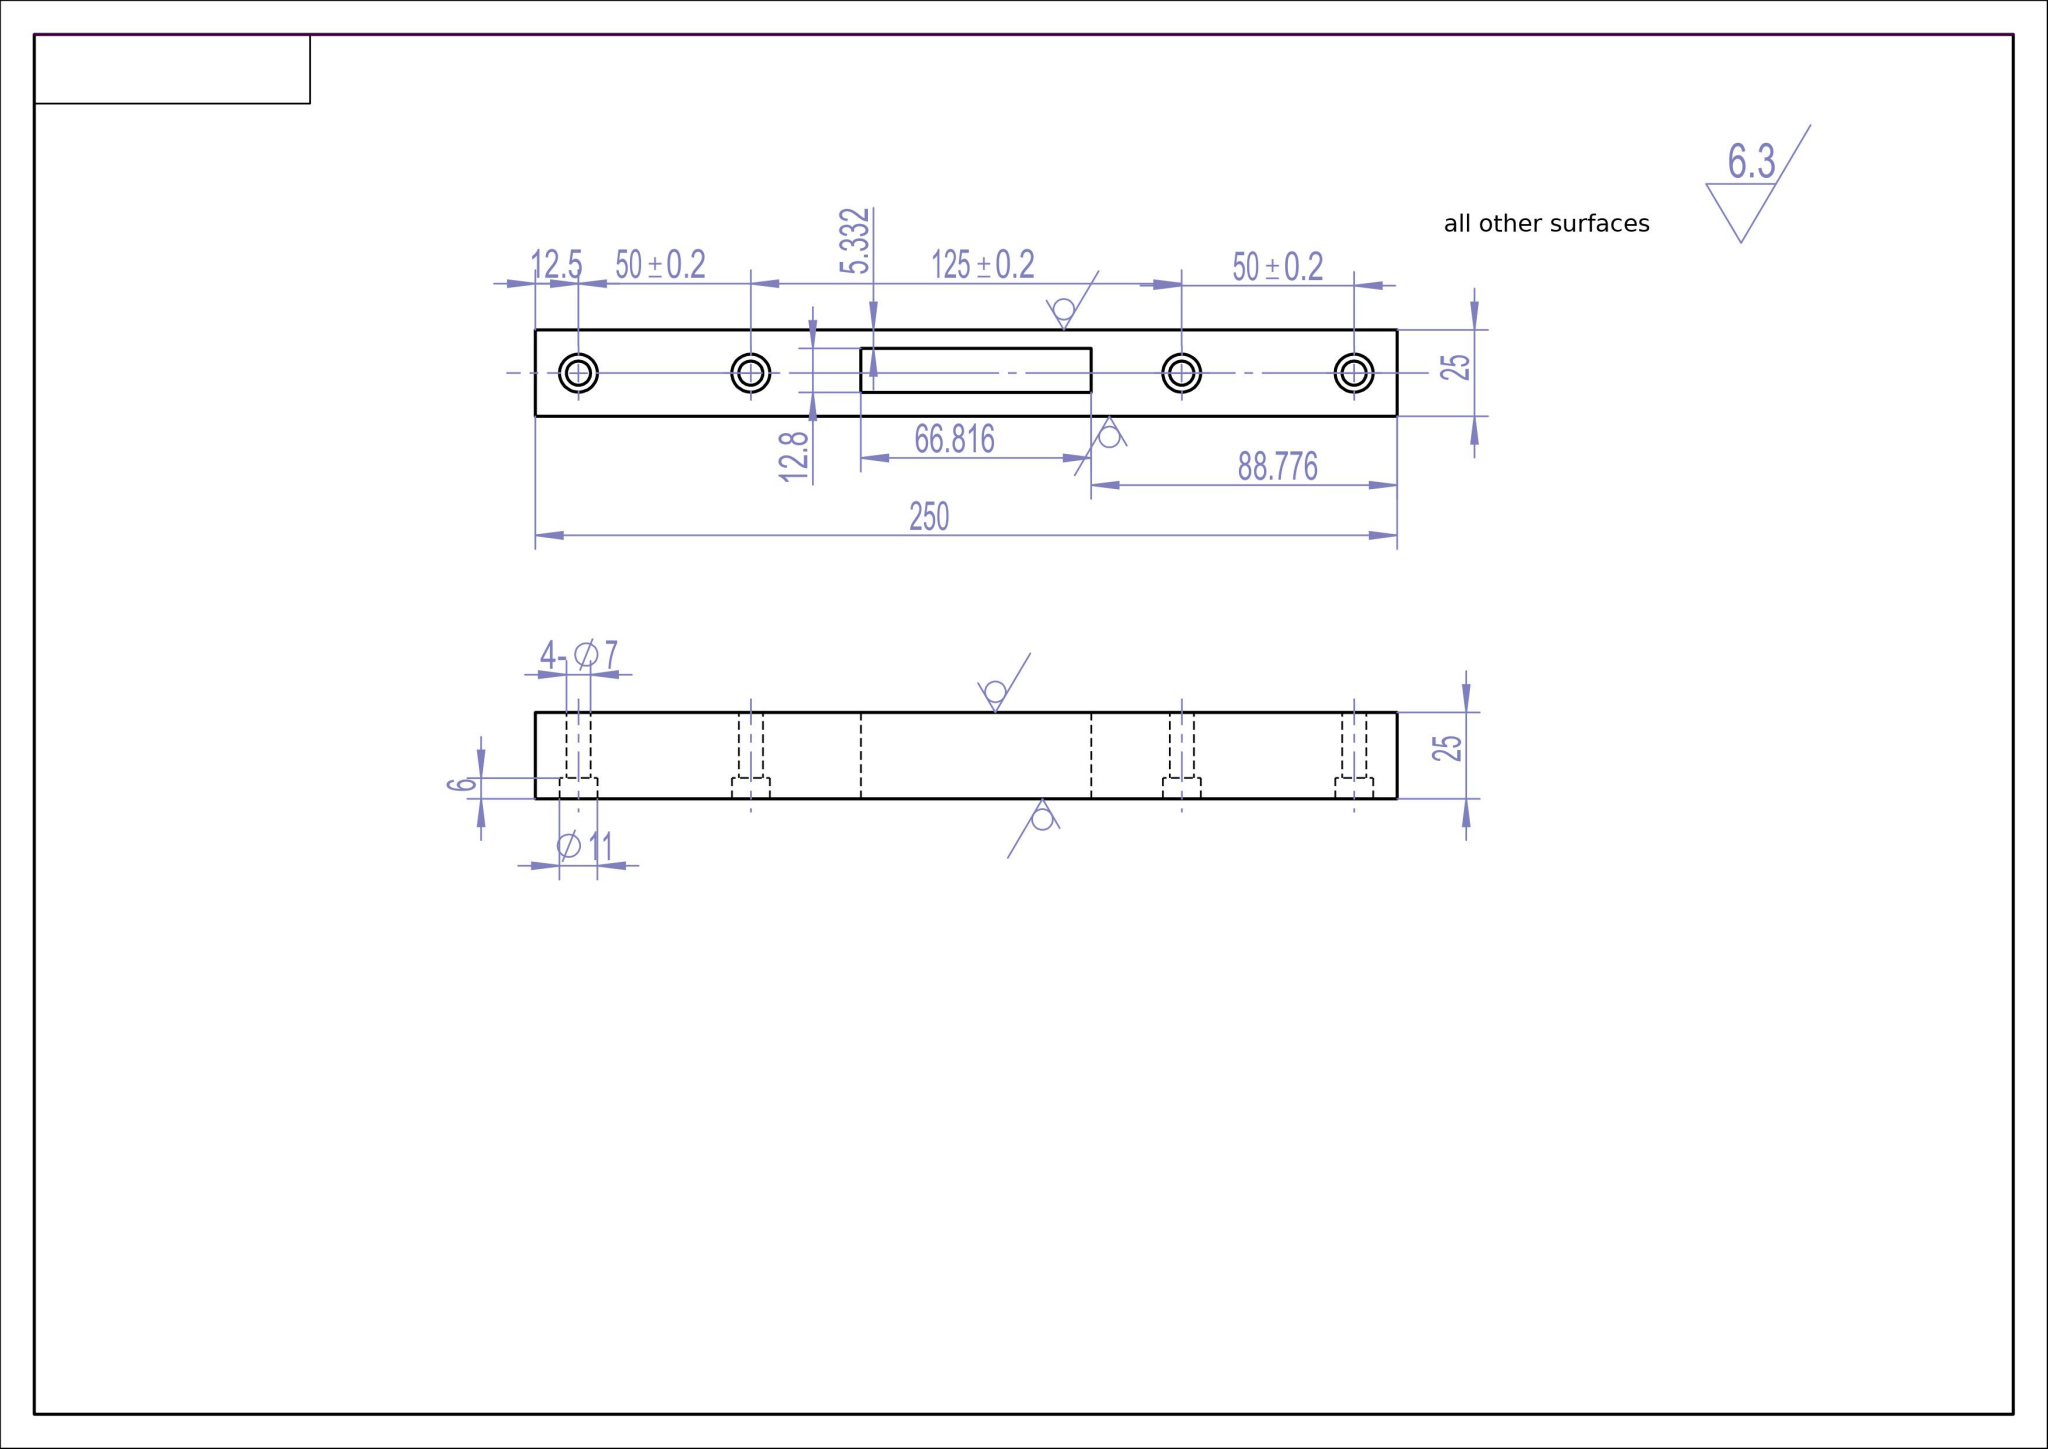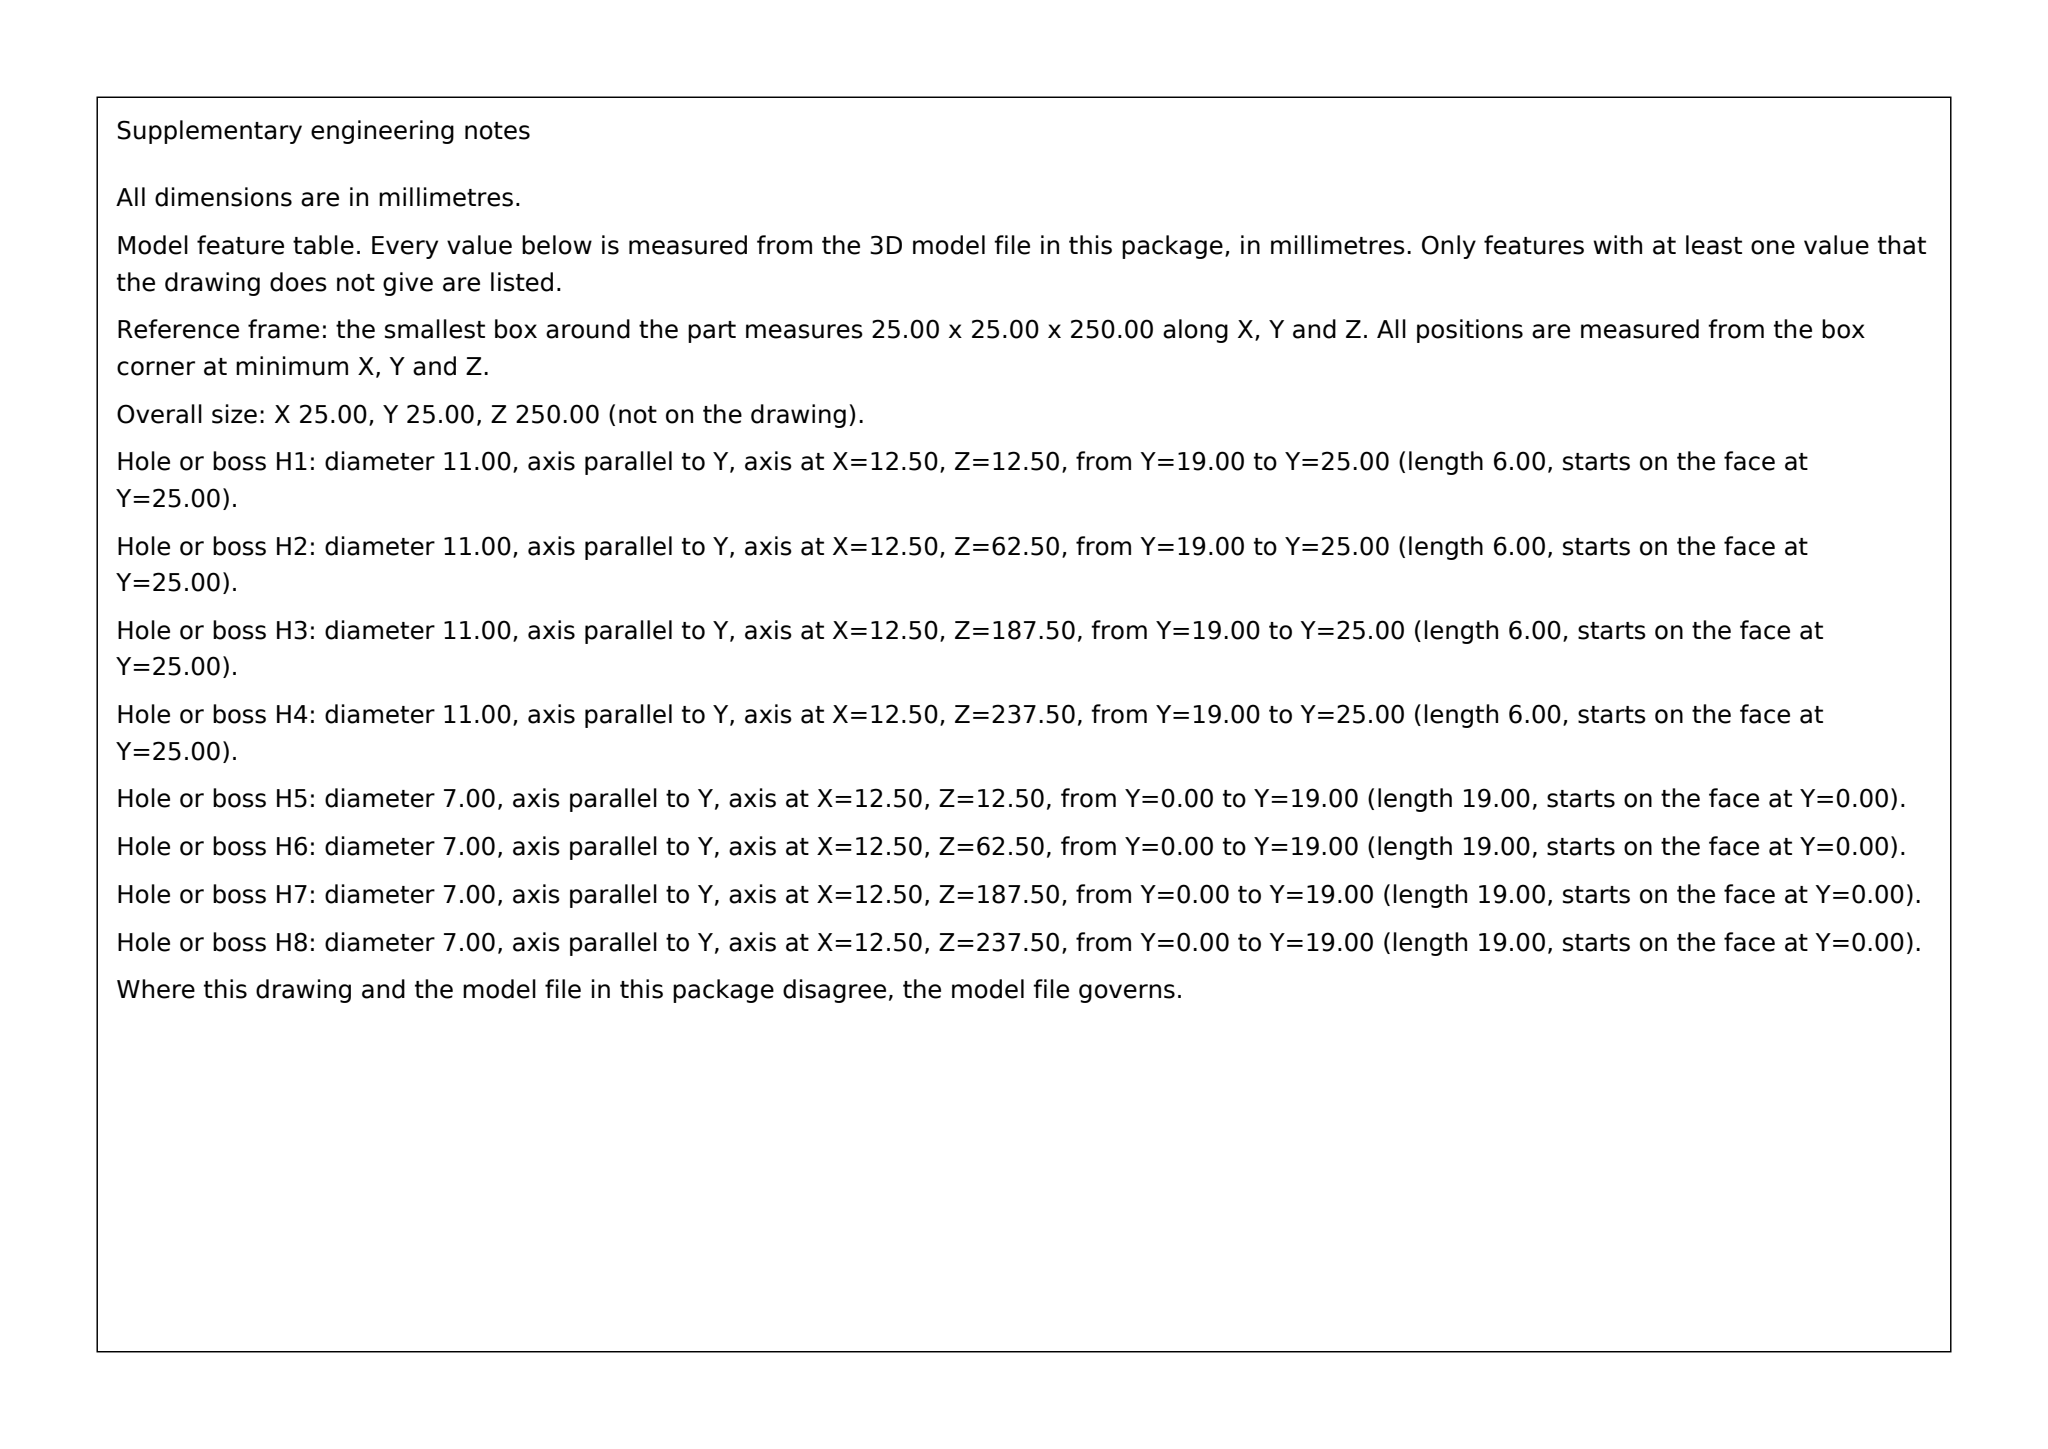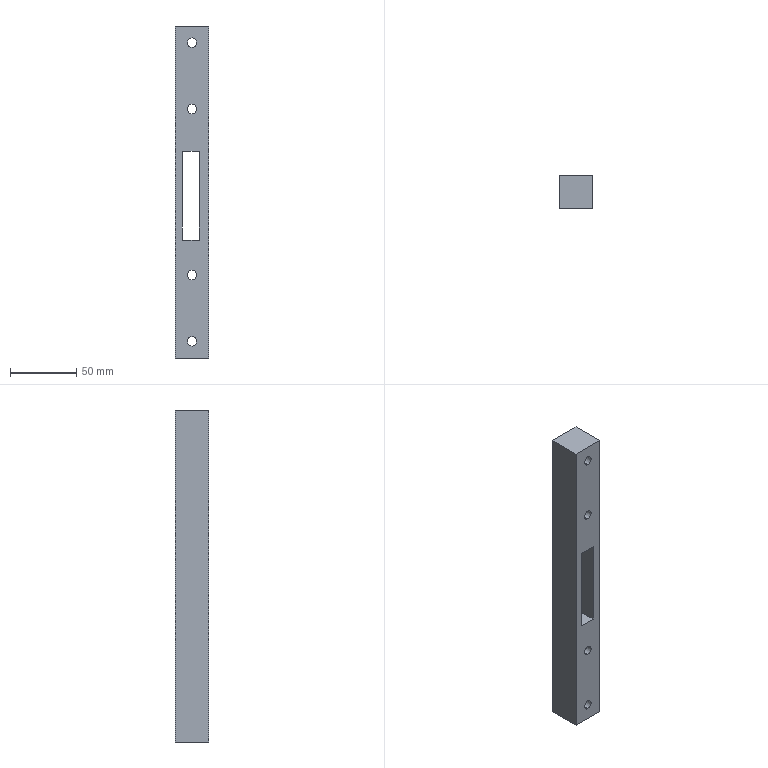Part | SolidWorks | mm | 1 solid | 30 faces | box 25 x 25 x 250 mm | volume 129663 mm3 | cylinder 16 | plane 14 | commonest cylinder face diameters 7 x8 11 x8
build123d program:
from build123d import *

# Parameters (mm, degrees)
SKETCH1_W                 = 25
SKETCH1_H                 = 25
BOSS_EXTRUDE1_DEPTH       = 250
SKETCH2_R                 = 5.5
CUT_EXTRUDE1_DEPTH        = 6
SKETCH3_R                 = 3.5
CUT_EXTRUDE2_DEPTH        = 26
LPATTERN1_COUNT           = 2
LPATTERN1_PITCH           = 50
LPATTERN2_COUNT           = 2
LPATTERN2_PITCH           = 175
LPATTERN2_COPY_1_SKETCH_R = 5.5
LPATTERN2_COPY_1_DEPTH    = 6
LPATTERN2_COPY_2_SKETCH_R = 3.5
LPATTERN2_COPY_2_DEPTH    = 26
SKETCH4_W                 = 12.8
SKETCH4_H                 = 66.816
CUT_EXTRUDE3_DEPTH        = 88


with BuildPart() as part:
    # Sketch1 → Boss-Extrude1 (new body)
    with BuildSketch(Plane.XY):
        with Locations((-44.867, 3.806)):
            Rectangle(SKETCH1_W, SKETCH1_H)
    extrude(amount=BOSS_EXTRUDE1_DEPTH)

    # Sketch2 → Cut-Extrude1 (cut)
    with BuildSketch(Plane(origin=(0, 16.306, 0), x_dir=(1, 0, 0), z_dir=(0, 1, 0))):
        with Locations(Location((-44.867, -12.5, 0), (0, 0, 270))):
            Circle(SKETCH2_R)
    cut_extrude1 = extrude(amount=-CUT_EXTRUDE1_DEPTH, mode=Mode.SUBTRACT)

    # Sketch3 → Cut-Extrude2 (cut)
    with BuildSketch(Plane(origin=(0, 10.306, 0), x_dir=(1, 0, 0), z_dir=(0, 1, 0))):
        with Locations(Location((-44.867, -12.5, 0), (0, 0, 270))):
            Circle(SKETCH3_R)
    cut_extrude2 = extrude(amount=-CUT_EXTRUDE2_DEPTH, mode=Mode.SUBTRACT)

    # LPattern1: Cut-Extrude1, Cut-Extrude2 ×2
    with Locations(*[(0, 0, i * LPATTERN1_PITCH) for i in range(1, LPATTERN1_COUNT)]):
        add(cut_extrude1, mode=Mode.SUBTRACT)
        add(cut_extrude2, mode=Mode.SUBTRACT)

    # LPattern2: Cut-Extrude1, Cut-Extrude2 ×2
    with Locations(*[(0, 0, i * LPATTERN2_PITCH) for i in range(1, LPATTERN2_COUNT)]):
        add(cut_extrude1, mode=Mode.SUBTRACT)
        add(cut_extrude2, mode=Mode.SUBTRACT)

    # LPattern2 copy 1 sketch → LPattern2 copy 1 (cut)
    with BuildSketch(Plane(origin=(0, 16.306, 225), x_dir=(1, 0, 0), z_dir=(0, 1, 0))):
        with Locations(Location((-44.867, -12.5, 0), (0, 0, 270))):
            Circle(LPATTERN2_COPY_1_SKETCH_R)
    extrude(amount=-LPATTERN2_COPY_1_DEPTH, mode=Mode.SUBTRACT)

    # LPattern2 copy 2 sketch → LPattern2 copy 2 (cut)
    with BuildSketch(Plane(origin=(0, 10.306, 225), x_dir=(1, 0, 0), z_dir=(0, 1, 0))):
        with Locations(Location((-44.867, -12.5, 0), (0, 0, 270))):
            Circle(LPATTERN2_COPY_2_SKETCH_R)
    extrude(amount=-LPATTERN2_COPY_2_DEPTH, mode=Mode.SUBTRACT)

    # Sketch4 → Cut-Extrude3 (cut)
    with BuildSketch(Plane(origin=(0, 16.306, 0), x_dir=(1, 0, 0), z_dir=(0, 1, 0))):
        with Locations((-45.635, -122.184)):
            Rectangle(SKETCH4_W, SKETCH4_H)
    extrude(amount=-CUT_EXTRUDE3_DEPTH, mode=Mode.SUBTRACT)


solid = part.part
STEP:
#1=CARTESIAN_POINT('',(-44.867,-8.694,234.));
#2=VERTEX_POINT('',#1);
#3=CARTESIAN_POINT('',(-44.867,-8.694,241.));
#4=VERTEX_POINT('',#3);
#5=CARTESIAN_POINT('',(-44.867,-8.694,237.5));
#6=DIRECTION('',(0.,1.,0.));
#7=DIRECTION('',(0.,0.,1.));
#8=AXIS2_PLACEMENT_3D('',#5,#6,#7);
#9=CIRCLE('',#8,3.5);
#10=EDGE_CURVE('',#2,#4,#9,.T.);
#11=ORIENTED_EDGE('',*,*,#10,.F.);
#12=CARTESIAN_POINT('',(-44.867,10.306,234.));
#13=VERTEX_POINT('',#12);
#14=CARTESIAN_POINT('',(-44.867,-15.694,234.));
#15=DIRECTION('',(0.,1.,0.));
#16=VECTOR('',#15,1000.);
#17=LINE('',#14,#16);
#18=EDGE_CURVE('',#2,#13,#17,.T.);
#19=ORIENTED_EDGE('',*,*,#18,.T.);
#20=CARTESIAN_POINT('',(-44.867,10.306,241.));
#21=VERTEX_POINT('',#20);
#22=CARTESIAN_POINT('',(-44.867,10.306,237.5));
#23=DIRECTION('',(0.,1.,0.));
#24=DIRECTION('',(0.,0.,1.));
#25=AXIS2_PLACEMENT_3D('',#22,#23,#24);
#26=CIRCLE('',#25,3.5);
#27=EDGE_CURVE('',#13,#21,#26,.T.);
#28=ORIENTED_EDGE('',*,*,#27,.T.);
#29=CARTESIAN_POINT('',(-44.867,-15.694,241.));
#30=DIRECTION('',(0.,1.,0.));
#31=VECTOR('',#30,1000.);
#32=LINE('',#29,#31);
#33=EDGE_CURVE('',#4,#21,#32,.T.);
#34=ORIENTED_EDGE('',*,*,#33,.F.);
#35=EDGE_LOOP('',(#11,#19,#28,#34));
#36=FACE_OUTER_BOUND('',#35,.T.);
#37=CARTESIAN_POINT('',(-44.867,-15.694,237.5));
#38=DIRECTION('',(0.,1.,0.));
#39=DIRECTION('',(0.,0.,1.));
#40=AXIS2_PLACEMENT_3D('',#37,#38,#39);
#41=CYLINDRICAL_SURFACE('',#40,3.5);
#42=ADVANCED_FACE('',(#36),#41,.F.);
#43=CARTESIAN_POINT('',(-44.867,-8.694,184.));
#44=VERTEX_POINT('',#43);
#45=CARTESIAN_POINT('',(-44.867,-8.694,191.));
#46=VERTEX_POINT('',#45);
#47=CARTESIAN_POINT('',(-44.867,-8.694,187.5));
#48=DIRECTION('',(0.,1.,0.));
#49=DIRECTION('',(0.,0.,1.));
#50=AXIS2_PLACEMENT_3D('',#47,#48,#49);
#51=CIRCLE('',#50,3.5);
#52=EDGE_CURVE('',#44,#46,#51,.T.);
#53=ORIENTED_EDGE('',*,*,#52,.F.);
#54=CARTESIAN_POINT('',(-44.867,10.306,184.));
#55=VERTEX_POINT('',#54);
#56=CARTESIAN_POINT('',(-44.867,-15.694,184.));
#57=DIRECTION('',(0.,1.,0.));
#58=VECTOR('',#57,1000.);
#59=LINE('',#56,#58);
#60=EDGE_CURVE('',#44,#55,#59,.T.);
#61=ORIENTED_EDGE('',*,*,#60,.T.);
#62=CARTESIAN_POINT('',(-44.867,10.306,191.));
#63=VERTEX_POINT('',#62);
#64=CARTESIAN_POINT('',(-44.867,10.306,187.5));
#65=DIRECTION('',(0.,1.,0.));
#66=DIRECTION('',(0.,0.,1.));
#67=AXIS2_PLACEMENT_3D('',#64,#65,#66);
#68=CIRCLE('',#67,3.5);
#69=EDGE_CURVE('',#55,#63,#68,.T.);
#70=ORIENTED_EDGE('',*,*,#69,.T.);
#71=CARTESIAN_POINT('',(-44.867,-15.694,191.));
#72=DIRECTION('',(0.,1.,0.));
#73=VECTOR('',#72,1000.);
#74=LINE('',#71,#73);
#75=EDGE_CURVE('',#46,#63,#74,.T.);
#76=ORIENTED_EDGE('',*,*,#75,.F.);
#77=EDGE_LOOP('',(#53,#61,#70,#76));
#78=FACE_OUTER_BOUND('',#77,.T.);
#79=CARTESIAN_POINT('',(-44.867,-15.694,187.5));
#80=DIRECTION('',(0.,1.,0.));
#81=DIRECTION('',(0.,0.,1.));
#82=AXIS2_PLACEMENT_3D('',#79,#80,#81);
#83=CYLINDRICAL_SURFACE('',#82,3.5);
#84=ADVANCED_FACE('',(#78),#83,.F.);
#85=CARTESIAN_POINT('',(-44.867,10.306,232.));
#86=VERTEX_POINT('',#85);
#87=CARTESIAN_POINT('',(-44.867,10.306,243.));
#88=VERTEX_POINT('',#87);
#89=CARTESIAN_POINT('',(-44.867,10.306,237.5));
#90=DIRECTION('',(0.,1.,0.));
#91=DIRECTION('',(0.,0.,1.));
#92=AXIS2_PLACEMENT_3D('',#89,#90,#91);
#93=CIRCLE('',#92,5.5);
#94=EDGE_CURVE('',#86,#88,#93,.T.);
#95=ORIENTED_EDGE('',*,*,#94,.F.);
#96=CARTESIAN_POINT('',(-44.867,16.306,232.));
#97=VERTEX_POINT('',#96);
#98=CARTESIAN_POINT('',(-44.867,10.306,232.));
#99=DIRECTION('',(0.,1.,0.));
#100=VECTOR('',#99,1000.);
#101=LINE('',#98,#100);
#102=EDGE_CURVE('',#86,#97,#101,.T.);
#103=ORIENTED_EDGE('',*,*,#102,.T.);
#104=CARTESIAN_POINT('',(-44.867,16.306,243.));
#105=VERTEX_POINT('',#104);
#106=CARTESIAN_POINT('',(-44.867,16.306,237.5));
#107=DIRECTION('',(0.,1.,0.));
#108=DIRECTION('',(0.,0.,1.));
#109=AXIS2_PLACEMENT_3D('',#106,#107,#108);
#110=CIRCLE('',#109,5.5);
#111=EDGE_CURVE('',#97,#105,#110,.T.);
#112=ORIENTED_EDGE('',*,*,#111,.T.);
#113=CARTESIAN_POINT('',(-44.867,10.306,243.));
#114=DIRECTION('',(0.,1.,0.));
#115=VECTOR('',#114,1000.);
#116=LINE('',#113,#115);
#117=EDGE_CURVE('',#88,#105,#116,.T.);
#118=ORIENTED_EDGE('',*,*,#117,.F.);
#119=EDGE_LOOP('',(#95,#103,#112,#118));
#120=FACE_OUTER_BOUND('',#119,.T.);
#121=CARTESIAN_POINT('',(-44.867,10.306,237.5));
#122=DIRECTION('',(0.,1.,0.));
#123=DIRECTION('',(0.,0.,1.));
#124=AXIS2_PLACEMENT_3D('',#121,#122,#123);
#125=CYLINDRICAL_SURFACE('',#124,5.5);
#126=ADVANCED_FACE('',(#120),#125,.F.);
#127=CARTESIAN_POINT('',(-44.867,10.306,182.));
#128=VERTEX_POINT('',#127);
#129=CARTESIAN_POINT('',(-44.867,10.306,193.));
#130=VERTEX_POINT('',#129);
#131=CARTESIAN_POINT('',(-44.867,10.306,187.5));
#132=DIRECTION('',(0.,1.,0.));
#133=DIRECTION('',(0.,0.,1.));
#134=AXIS2_PLACEMENT_3D('',#131,#132,#133);
#135=CIRCLE('',#134,5.5);
#136=EDGE_CURVE('',#128,#130,#135,.T.);
#137=ORIENTED_EDGE('',*,*,#136,.F.);
#138=CARTESIAN_POINT('',(-44.867,16.306,182.));
#139=VERTEX_POINT('',#138);
#140=CARTESIAN_POINT('',(-44.867,10.306,182.));
#141=DIRECTION('',(0.,1.,0.));
#142=VECTOR('',#141,1000.);
#143=LINE('',#140,#142);
#144=EDGE_CURVE('',#128,#139,#143,.T.);
#145=ORIENTED_EDGE('',*,*,#144,.T.);
#146=CARTESIAN_POINT('',(-44.867,16.306,193.));
#147=VERTEX_POINT('',#146);
#148=CARTESIAN_POINT('',(-44.867,16.306,187.5));
#149=DIRECTION('',(0.,1.,0.));
#150=DIRECTION('',(0.,0.,1.));
#151=AXIS2_PLACEMENT_3D('',#148,#149,#150);
#152=CIRCLE('',#151,5.5);
#153=EDGE_CURVE('',#139,#147,#152,.T.);
#154=ORIENTED_EDGE('',*,*,#153,.T.);
#155=CARTESIAN_POINT('',(-44.867,10.306,193.));
#156=DIRECTION('',(0.,1.,0.));
#157=VECTOR('',#156,1000.);
#158=LINE('',#155,#157);
#159=EDGE_CURVE('',#130,#147,#158,.T.);
#160=ORIENTED_EDGE('',*,*,#159,.F.);
#161=EDGE_LOOP('',(#137,#145,#154,#160));
#162=FACE_OUTER_BOUND('',#161,.T.);
#163=CARTESIAN_POINT('',(-44.867,10.306,187.5));
#164=DIRECTION('',(0.,1.,0.));
#165=DIRECTION('',(0.,0.,1.));
#166=AXIS2_PLACEMENT_3D('',#163,#164,#165);
#167=CYLINDRICAL_SURFACE('',#166,5.5);
#168=ADVANCED_FACE('',(#162),#167,.F.);
#169=CARTESIAN_POINT('',(-44.867,-8.694,59.));
#170=VERTEX_POINT('',#169);
#171=CARTESIAN_POINT('',(-44.867,-8.694,66.));
#172=VERTEX_POINT('',#171);
#173=CARTESIAN_POINT('',(-44.867,-8.694,62.5));
#174=DIRECTION('',(0.,1.,0.));
#175=DIRECTION('',(0.,0.,1.));
#176=AXIS2_PLACEMENT_3D('',#173,#174,#175);
#177=CIRCLE('',#176,3.5);
#178=EDGE_CURVE('',#170,#172,#177,.T.);
#179=ORIENTED_EDGE('',*,*,#178,.F.);
#180=CARTESIAN_POINT('',(-44.867,10.306,59.));
#181=VERTEX_POINT('',#180);
#182=CARTESIAN_POINT('',(-44.867,-15.694,59.));
#183=DIRECTION('',(0.,1.,0.));
#184=VECTOR('',#183,1000.);
#185=LINE('',#182,#184);
#186=EDGE_CURVE('',#170,#181,#185,.T.);
#187=ORIENTED_EDGE('',*,*,#186,.T.);
#188=CARTESIAN_POINT('',(-44.867,10.306,66.));
#189=VERTEX_POINT('',#188);
#190=CARTESIAN_POINT('',(-44.867,10.306,62.5));
#191=DIRECTION('',(0.,1.,0.));
#192=DIRECTION('',(0.,0.,1.));
#193=AXIS2_PLACEMENT_3D('',#190,#191,#192);
#194=CIRCLE('',#193,3.5);
#195=EDGE_CURVE('',#181,#189,#194,.T.);
#196=ORIENTED_EDGE('',*,*,#195,.T.);
#197=CARTESIAN_POINT('',(-44.867,-15.694,66.));
#198=DIRECTION('',(0.,1.,0.));
#199=VECTOR('',#198,1000.);
#200=LINE('',#197,#199);
#201=EDGE_CURVE('',#172,#189,#200,.T.);
#202=ORIENTED_EDGE('',*,*,#201,.F.);
#203=EDGE_LOOP('',(#179,#187,#196,#202));
#204=FACE_OUTER_BOUND('',#203,.T.);
#205=CARTESIAN_POINT('',(-44.867,-15.694,62.5));
#206=DIRECTION('',(0.,1.,0.));
#207=DIRECTION('',(0.,0.,1.));
#208=AXIS2_PLACEMENT_3D('',#205,#206,#207);
#209=CYLINDRICAL_SURFACE('',#208,3.5);
#210=ADVANCED_FACE('',(#204),#209,.F.);
#211=CARTESIAN_POINT('',(-44.867,10.306,57.));
#212=VERTEX_POINT('',#211);
#213=CARTESIAN_POINT('',(-44.867,10.306,68.));
#214=VERTEX_POINT('',#213);
#215=CARTESIAN_POINT('',(-44.867,10.306,62.5));
#216=DIRECTION('',(0.,1.,0.));
#217=DIRECTION('',(0.,0.,1.));
#218=AXIS2_PLACEMENT_3D('',#215,#216,#217);
#219=CIRCLE('',#218,5.5);
#220=EDGE_CURVE('',#212,#214,#219,.T.);
#221=ORIENTED_EDGE('',*,*,#220,.F.);
#222=CARTESIAN_POINT('',(-44.867,16.306,57.));
#223=VERTEX_POINT('',#222);
#224=CARTESIAN_POINT('',(-44.867,10.306,57.));
#225=DIRECTION('',(0.,1.,0.));
#226=VECTOR('',#225,1000.);
#227=LINE('',#224,#226);
#228=EDGE_CURVE('',#212,#223,#227,.T.);
#229=ORIENTED_EDGE('',*,*,#228,.T.);
#230=CARTESIAN_POINT('',(-44.867,16.306,68.));
#231=VERTEX_POINT('',#230);
#232=CARTESIAN_POINT('',(-44.867,16.306,62.5));
#233=DIRECTION('',(0.,1.,0.));
#234=DIRECTION('',(0.,0.,1.));
#235=AXIS2_PLACEMENT_3D('',#232,#233,#234);
#236=CIRCLE('',#235,5.5);
#237=EDGE_CURVE('',#223,#231,#236,.T.);
#238=ORIENTED_EDGE('',*,*,#237,.T.);
#239=CARTESIAN_POINT('',(-44.867,10.306,68.));
#240=DIRECTION('',(0.,1.,0.));
#241=VECTOR('',#240,1000.);
#242=LINE('',#239,#241);
#243=EDGE_CURVE('',#214,#231,#242,.T.);
#244=ORIENTED_EDGE('',*,*,#243,.F.);
#245=EDGE_LOOP('',(#221,#229,#238,#244));
#246=FACE_OUTER_BOUND('',#245,.T.);
#247=CARTESIAN_POINT('',(-44.867,10.306,62.5));
#248=DIRECTION('',(0.,1.,0.));
#249=DIRECTION('',(0.,0.,1.));
#250=AXIS2_PLACEMENT_3D('',#247,#248,#249);
#251=CYLINDRICAL_SURFACE('',#250,5.5);
#252=ADVANCED_FACE('',(#246),#251,.F.);
#253=CARTESIAN_POINT('',(-44.867,-8.694,9.));
#254=VERTEX_POINT('',#253);
#255=CARTESIAN_POINT('',(-44.867,-8.694,16.));
#256=VERTEX_POINT('',#255);
#257=CARTESIAN_POINT('',(-44.867,-8.694,12.5));
#258=DIRECTION('',(0.,1.,0.));
#259=DIRECTION('',(0.,0.,1.));
#260=AXIS2_PLACEMENT_3D('',#257,#258,#259);
#261=CIRCLE('',#260,3.5);
#262=EDGE_CURVE('',#254,#256,#261,.T.);
#263=ORIENTED_EDGE('',*,*,#262,.F.);
#264=CARTESIAN_POINT('',(-44.867,10.306,9.));
#265=VERTEX_POINT('',#264);
#266=CARTESIAN_POINT('',(-44.867,-15.694,9.));
#267=DIRECTION('',(0.,1.,0.));
#268=VECTOR('',#267,1000.);
#269=LINE('',#266,#268);
#270=EDGE_CURVE('',#254,#265,#269,.T.);
#271=ORIENTED_EDGE('',*,*,#270,.T.);
#272=CARTESIAN_POINT('',(-44.867,10.306,16.));
#273=VERTEX_POINT('',#272);
#274=CARTESIAN_POINT('',(-44.867,10.306,12.5));
#275=DIRECTION('',(0.,1.,0.));
#276=DIRECTION('',(0.,0.,1.));
#277=AXIS2_PLACEMENT_3D('',#274,#275,#276);
#278=CIRCLE('',#277,3.5);
#279=EDGE_CURVE('',#265,#273,#278,.T.);
#280=ORIENTED_EDGE('',*,*,#279,.T.);
#281=CARTESIAN_POINT('',(-44.867,-15.694,16.));
#282=DIRECTION('',(0.,1.,0.));
#283=VECTOR('',#282,1000.);
#284=LINE('',#281,#283);
#285=EDGE_CURVE('',#256,#273,#284,.T.);
#286=ORIENTED_EDGE('',*,*,#285,.F.);
#287=EDGE_LOOP('',(#263,#271,#280,#286));
#288=FACE_OUTER_BOUND('',#287,.T.);
#289=CARTESIAN_POINT('',(-44.867,-15.694,12.5));
#290=DIRECTION('',(0.,1.,0.));
#291=DIRECTION('',(0.,0.,1.));
#292=AXIS2_PLACEMENT_3D('',#289,#290,#291);
#293=CYLINDRICAL_SURFACE('',#292,3.5);
#294=ADVANCED_FACE('',(#288),#293,.F.);
#295=CARTESIAN_POINT('',(-44.867,10.306,7.));
#296=VERTEX_POINT('',#295);
#297=CARTESIAN_POINT('',(-44.867,10.306,18.));
#298=VERTEX_POINT('',#297);
#299=CARTESIAN_POINT('',(-44.867,10.306,12.5));
#300=DIRECTION('',(0.,1.,0.));
#301=DIRECTION('',(0.,0.,1.));
#302=AXIS2_PLACEMENT_3D('',#299,#300,#301);
#303=CIRCLE('',#302,5.5);
#304=EDGE_CURVE('',#296,#298,#303,.T.);
#305=ORIENTED_EDGE('',*,*,#304,.F.);
#306=CARTESIAN_POINT('',(-44.867,16.306,7.));
#307=VERTEX_POINT('',#306);
#308=CARTESIAN_POINT('',(-44.867,10.306,7.));
#309=DIRECTION('',(0.,1.,0.));
#310=VECTOR('',#309,1000.);
#311=LINE('',#308,#310);
#312=EDGE_CURVE('',#296,#307,#311,.T.);
#313=ORIENTED_EDGE('',*,*,#312,.T.);
#314=CARTESIAN_POINT('',(-44.867,16.306,18.));
#315=VERTEX_POINT('',#314);
#316=CARTESIAN_POINT('',(-44.867,16.306,12.5));
#317=DIRECTION('',(0.,1.,0.));
#318=DIRECTION('',(0.,0.,1.));
#319=AXIS2_PLACEMENT_3D('',#316,#317,#318);
#320=CIRCLE('',#319,5.5);
#321=EDGE_CURVE('',#307,#315,#320,.T.);
#322=ORIENTED_EDGE('',*,*,#321,.T.);
#323=CARTESIAN_POINT('',(-44.867,10.306,18.));
#324=DIRECTION('',(0.,1.,0.));
#325=VECTOR('',#324,1000.);
#326=LINE('',#323,#325);
#327=EDGE_CURVE('',#298,#315,#326,.T.);
#328=ORIENTED_EDGE('',*,*,#327,.F.);
#329=EDGE_LOOP('',(#305,#313,#322,#328));
#330=FACE_OUTER_BOUND('',#329,.T.);
#331=CARTESIAN_POINT('',(-44.867,10.306,12.5));
#332=DIRECTION('',(0.,1.,0.));
#333=DIRECTION('',(0.,0.,1.));
#334=AXIS2_PLACEMENT_3D('',#331,#332,#333);
#335=CYLINDRICAL_SURFACE('',#334,5.5);
#336=ADVANCED_FACE('',(#330),#335,.F.);
#337=CARTESIAN_POINT('',(-57.367,16.306,0.));
#338=VERTEX_POINT('',#337);
#339=CARTESIAN_POINT('',(-57.367,-8.694,0.));
#340=VERTEX_POINT('',#339);
#341=CARTESIAN_POINT('',(-57.367,16.306,0.));
#342=DIRECTION('',(0.,-1.,0.));
#343=VECTOR('',#342,1000.);
#344=LINE('',#341,#343);
#345=EDGE_CURVE('',#338,#340,#344,.T.);
#346=ORIENTED_EDGE('',*,*,#345,.T.);
#347=CARTESIAN_POINT('',(-57.367,-8.694,250.));
#348=VERTEX_POINT('',#347);
#349=CARTESIAN_POINT('',(-57.367,-8.694,250.));
#350=DIRECTION('',(0.,0.,-1.));
#351=VECTOR('',#350,1000.);
#352=LINE('',#349,#351);
#353=EDGE_CURVE('',#348,#340,#352,.T.);
#354=ORIENTED_EDGE('',*,*,#353,.F.);
#355=CARTESIAN_POINT('',(-57.367,16.306,250.));
#356=VERTEX_POINT('',#355);
#357=CARTESIAN_POINT('',(-57.367,16.306,250.));
#358=DIRECTION('',(0.,-1.,0.));
#359=VECTOR('',#358,1000.);
#360=LINE('',#357,#359);
#361=EDGE_CURVE('',#356,#348,#360,.T.);
#362=ORIENTED_EDGE('',*,*,#361,.F.);
#363=CARTESIAN_POINT('',(-57.367,16.306,250.));
#364=DIRECTION('',(0.,0.,-1.));
#365=VECTOR('',#364,1000.);
#366=LINE('',#363,#365);
#367=EDGE_CURVE('',#356,#338,#366,.T.);
#368=ORIENTED_EDGE('',*,*,#367,.T.);
#369=EDGE_LOOP('',(#346,#354,#362,#368));
#370=FACE_OUTER_BOUND('',#369,.T.);
#371=CARTESIAN_POINT('',(-57.367,16.306,250.));
#372=DIRECTION('',(1.,0.,0.));
#373=DIRECTION('',(-0.,1.,0.));
#374=AXIS2_PLACEMENT_3D('',#371,#372,#373);
#375=PLANE('',#374);
#376=ADVANCED_FACE('',(#370),#375,.F.);
#377=CARTESIAN_POINT('',(-39.235,-8.694,88.776));
#378=VERTEX_POINT('',#377);
#379=CARTESIAN_POINT('',(-52.035,-8.694,88.776));
#380=VERTEX_POINT('',#379);
#381=CARTESIAN_POINT('',(-57.367,-8.694,88.776));
#382=DIRECTION('',(-1.,0.,0.));
#383=VECTOR('',#382,1000.);
#384=LINE('',#381,#383);
#385=EDGE_CURVE('',#378,#380,#384,.T.);
#386=ORIENTED_EDGE('',*,*,#385,.T.);
#387=CARTESIAN_POINT('',(-52.035,-8.694,155.592));
#388=VERTEX_POINT('',#387);
#389=CARTESIAN_POINT('',(-52.035,-8.694,250.));
#390=DIRECTION('',(0.,0.,1.));
#391=VECTOR('',#390,1000.);
#392=LINE('',#389,#391);
#393=EDGE_CURVE('',#380,#388,#392,.T.);
#394=ORIENTED_EDGE('',*,*,#393,.T.);
#395=CARTESIAN_POINT('',(-39.235,-8.694,155.592));
#396=VERTEX_POINT('',#395);
#397=CARTESIAN_POINT('',(-57.367,-8.694,155.592));
#398=DIRECTION('',(1.,0.,0.));
#399=VECTOR('',#398,1000.);
#400=LINE('',#397,#399);
#401=EDGE_CURVE('',#388,#396,#400,.T.);
#402=ORIENTED_EDGE('',*,*,#401,.T.);
#403=CARTESIAN_POINT('',(-39.235,-8.694,250.));
#404=DIRECTION('',(0.,0.,-1.));
#405=VECTOR('',#404,1000.);
#406=LINE('',#403,#405);
#407=EDGE_CURVE('',#396,#378,#406,.T.);
#408=ORIENTED_EDGE('',*,*,#407,.T.);
#409=EDGE_LOOP('',(#386,#394,#402,#408));
#410=FACE_BOUND('',#409,.T.);
#411=CARTESIAN_POINT('',(-44.867,-8.694,237.5));
#412=DIRECTION('',(0.,1.,0.));
#413=DIRECTION('',(0.,0.,1.));
#414=AXIS2_PLACEMENT_3D('',#411,#412,#413);
#415=CIRCLE('',#414,3.5);
#416=EDGE_CURVE('',#4,#2,#415,.T.);
#417=ORIENTED_EDGE('',*,*,#416,.T.);
#418=ORIENTED_EDGE('',*,*,#10,.T.);
#419=EDGE_LOOP('',(#417,#418));
#420=FACE_BOUND('',#419,.T.);
#421=CARTESIAN_POINT('',(-44.867,-8.694,187.5));
#422=DIRECTION('',(0.,1.,0.));
#423=DIRECTION('',(0.,0.,1.));
#424=AXIS2_PLACEMENT_3D('',#421,#422,#423);
#425=CIRCLE('',#424,3.5);
#426=EDGE_CURVE('',#46,#44,#425,.T.);
#427=ORIENTED_EDGE('',*,*,#426,.T.);
#428=ORIENTED_EDGE('',*,*,#52,.T.);
#429=EDGE_LOOP('',(#427,#428));
#430=FACE_BOUND('',#429,.T.);
#431=CARTESIAN_POINT('',(-44.867,-8.694,62.5));
#432=DIRECTION('',(0.,1.,0.));
#433=DIRECTION('',(0.,0.,1.));
#434=AXIS2_PLACEMENT_3D('',#431,#432,#433);
#435=CIRCLE('',#434,3.5);
#436=EDGE_CURVE('',#172,#170,#435,.T.);
#437=ORIENTED_EDGE('',*,*,#436,.T.);
#438=ORIENTED_EDGE('',*,*,#178,.T.);
#439=EDGE_LOOP('',(#437,#438));
#440=FACE_BOUND('',#439,.T.);
#441=CARTESIAN_POINT('',(-44.867,-8.694,12.5));
#442=DIRECTION('',(0.,1.,0.));
#443=DIRECTION('',(0.,0.,1.));
#444=AXIS2_PLACEMENT_3D('',#441,#442,#443);
#445=CIRCLE('',#444,3.5);
#446=EDGE_CURVE('',#256,#254,#445,.T.);
#447=ORIENTED_EDGE('',*,*,#446,.T.);
#448=ORIENTED_EDGE('',*,*,#262,.T.);
#449=EDGE_LOOP('',(#447,#448));
#450=FACE_BOUND('',#449,.T.);
#451=CARTESIAN_POINT('',(-32.367,-8.694,0.));
#452=VERTEX_POINT('',#451);
#453=CARTESIAN_POINT('',(-57.367,-8.694,0.));
#454=DIRECTION('',(1.,0.,0.));
#455=VECTOR('',#454,1000.);
#456=LINE('',#453,#455);
#457=EDGE_CURVE('',#340,#452,#456,.T.);
#458=ORIENTED_EDGE('',*,*,#457,.T.);
#459=CARTESIAN_POINT('',(-32.367,-8.694,250.));
#460=VERTEX_POINT('',#459);
#461=CARTESIAN_POINT('',(-32.367,-8.694,250.));
#462=DIRECTION('',(0.,0.,-1.));
#463=VECTOR('',#462,1000.);
#464=LINE('',#461,#463);
#465=EDGE_CURVE('',#460,#452,#464,.T.);
#466=ORIENTED_EDGE('',*,*,#465,.F.);
#467=CARTESIAN_POINT('',(-57.367,-8.694,250.));
#468=DIRECTION('',(1.,0.,0.));
#469=VECTOR('',#468,1000.);
#470=LINE('',#467,#469);
#471=EDGE_CURVE('',#348,#460,#470,.T.);
#472=ORIENTED_EDGE('',*,*,#471,.F.);
#473=ORIENTED_EDGE('',*,*,#353,.T.);
#474=EDGE_LOOP('',(#458,#466,#472,#473));
#475=FACE_OUTER_BOUND('',#474,.T.);
#476=CARTESIAN_POINT('',(-57.367,-8.694,250.));
#477=DIRECTION('',(0.,1.,0.));
#478=DIRECTION('',(0.,0.,1.));
#479=AXIS2_PLACEMENT_3D('',#476,#477,#478);
#480=PLANE('',#479);
#481=ADVANCED_FACE('',(#410,#420,#430,#440,#450,#475),#480,.F.);
#482=CARTESIAN_POINT('',(-32.367,16.306,0.));
#483=VERTEX_POINT('',#482);
#484=CARTESIAN_POINT('',(-32.367,16.306,0.));
#485=DIRECTION('',(-0.,1.,0.));
#486=VECTOR('',#485,1000.);
#487=LINE('',#484,#486);
#488=EDGE_CURVE('',#452,#483,#487,.T.);
#489=ORIENTED_EDGE('',*,*,#488,.T.);
#490=CARTESIAN_POINT('',(-32.367,16.306,250.));
#491=VERTEX_POINT('',#490);
#492=CARTESIAN_POINT('',(-32.367,16.306,250.));
#493=DIRECTION('',(0.,0.,-1.));
#494=VECTOR('',#493,1000.);
#495=LINE('',#492,#494);
#496=EDGE_CURVE('',#491,#483,#495,.T.);
#497=ORIENTED_EDGE('',*,*,#496,.F.);
#498=CARTESIAN_POINT('',(-32.367,16.306,250.));
#499=DIRECTION('',(-0.,1.,0.));
#500=VECTOR('',#499,1000.);
#501=LINE('',#498,#500);
#502=EDGE_CURVE('',#460,#491,#501,.T.);
#503=ORIENTED_EDGE('',*,*,#502,.F.);
#504=ORIENTED_EDGE('',*,*,#465,.T.);
#505=EDGE_LOOP('',(#489,#497,#503,#504));
#506=FACE_OUTER_BOUND('',#505,.T.);
#507=CARTESIAN_POINT('',(-32.367,16.306,250.));
#508=DIRECTION('',(-1.,-0.,0.));
#509=DIRECTION('',(0.,-1.,0.));
#510=AXIS2_PLACEMENT_3D('',#507,#508,#509);
#511=PLANE('',#510);
#512=ADVANCED_FACE('',(#506),#511,.F.);
#513=CARTESIAN_POINT('',(-52.035,16.306,155.592));
#514=VERTEX_POINT('',#513);
#515=CARTESIAN_POINT('',(-39.235,16.306,155.592));
#516=VERTEX_POINT('',#515);
#517=CARTESIAN_POINT('',(-52.035,16.306,155.592));
#518=DIRECTION('',(1.,0.,0.));
#519=VECTOR('',#518,1000.);
#520=LINE('',#517,#519);
#521=EDGE_CURVE('',#514,#516,#520,.T.);
#522=ORIENTED_EDGE('',*,*,#521,.F.);
#523=CARTESIAN_POINT('',(-52.035,16.306,88.776));
#524=VERTEX_POINT('',#523);
#525=CARTESIAN_POINT('',(-52.035,16.306,88.776));
#526=DIRECTION('',(0.,0.,1.));
#527=VECTOR('',#526,1000.);
#528=LINE('',#525,#527);
#529=EDGE_CURVE('',#524,#514,#528,.T.);
#530=ORIENTED_EDGE('',*,*,#529,.F.);
#531=CARTESIAN_POINT('',(-39.235,16.306,88.776));
#532=VERTEX_POINT('',#531);
#533=CARTESIAN_POINT('',(-52.035,16.306,88.776));
#534=DIRECTION('',(-1.,0.,0.));
#535=VECTOR('',#534,1000.);
#536=LINE('',#533,#535);
#537=EDGE_CURVE('',#532,#524,#536,.T.);
#538=ORIENTED_EDGE('',*,*,#537,.F.);
#539=CARTESIAN_POINT('',(-39.235,16.306,88.776));
#540=DIRECTION('',(0.,0.,-1.));
#541=VECTOR('',#540,1000.);
#542=LINE('',#539,#541);
#543=EDGE_CURVE('',#516,#532,#542,.T.);
#544=ORIENTED_EDGE('',*,*,#543,.F.);
#545=EDGE_LOOP('',(#522,#530,#538,#544));
#546=FACE_BOUND('',#545,.T.);
#547=CARTESIAN_POINT('',(-44.867,16.306,237.5));
#548=DIRECTION('',(0.,1.,0.));
#549=DIRECTION('',(0.,0.,1.));
#550=AXIS2_PLACEMENT_3D('',#547,#548,#549);
#551=CIRCLE('',#550,5.5);
#552=EDGE_CURVE('',#105,#97,#551,.T.);
#553=ORIENTED_EDGE('',*,*,#552,.F.);
#554=ORIENTED_EDGE('',*,*,#111,.F.);
#555=EDGE_LOOP('',(#553,#554));
#556=FACE_BOUND('',#555,.T.);
#557=CARTESIAN_POINT('',(-44.867,16.306,187.5));
#558=DIRECTION('',(0.,1.,0.));
#559=DIRECTION('',(0.,0.,1.));
#560=AXIS2_PLACEMENT_3D('',#557,#558,#559);
#561=CIRCLE('',#560,5.5);
#562=EDGE_CURVE('',#147,#139,#561,.T.);
#563=ORIENTED_EDGE('',*,*,#562,.F.);
#564=ORIENTED_EDGE('',*,*,#153,.F.);
#565=EDGE_LOOP('',(#563,#564));
#566=FACE_BOUND('',#565,.T.);
#567=CARTESIAN_POINT('',(-44.867,16.306,62.5));
#568=DIRECTION('',(0.,1.,0.));
#569=DIRECTION('',(0.,0.,1.));
#570=AXIS2_PLACEMENT_3D('',#567,#568,#569);
#571=CIRCLE('',#570,5.5);
#572=EDGE_CURVE('',#231,#223,#571,.T.);
#573=ORIENTED_EDGE('',*,*,#572,.F.);
#574=ORIENTED_EDGE('',*,*,#237,.F.);
#575=EDGE_LOOP('',(#573,#574));
#576=FACE_BOUND('',#575,.T.);
#577=CARTESIAN_POINT('',(-44.867,16.306,12.5));
#578=DIRECTION('',(0.,1.,0.));
#579=DIRECTION('',(0.,0.,1.));
#580=AXIS2_PLACEMENT_3D('',#577,#578,#579);
#581=CIRCLE('',#580,5.5);
#582=EDGE_CURVE('',#315,#307,#581,.T.);
#583=ORIENTED_EDGE('',*,*,#582,.F.);
#584=ORIENTED_EDGE('',*,*,#321,.F.);
#585=EDGE_LOOP('',(#583,#584));
#586=FACE_BOUND('',#585,.T.);
#587=CARTESIAN_POINT('',(-57.367,16.306,0.));
#588=DIRECTION('',(-1.,0.,0.));
#589=VECTOR('',#588,1000.);
#590=LINE('',#587,#589);
#591=EDGE_CURVE('',#483,#338,#590,.T.);
#592=ORIENTED_EDGE('',*,*,#591,.T.);
#593=ORIENTED_EDGE('',*,*,#367,.F.);
#594=CARTESIAN_POINT('',(-57.367,16.306,250.));
#595=DIRECTION('',(-1.,0.,0.));
#596=VECTOR('',#595,1000.);
#597=LINE('',#594,#596);
#598=EDGE_CURVE('',#491,#356,#597,.T.);
#599=ORIENTED_EDGE('',*,*,#598,.F.);
#600=ORIENTED_EDGE('',*,*,#496,.T.);
#601=EDGE_LOOP('',(#592,#593,#599,#600));
#602=FACE_OUTER_BOUND('',#601,.T.);
#603=CARTESIAN_POINT('',(-57.367,16.306,250.));
#604=DIRECTION('',(0.,-1.,0.));
#605=DIRECTION('',(0.,0.,-1.));
#606=AXIS2_PLACEMENT_3D('',#603,#604,#605);
#607=PLANE('',#606);
#608=ADVANCED_FACE('',(#546,#556,#566,#576,#586,#602),#607,.F.);
#609=ORIENTED_EDGE('',*,*,#361,.T.);
#610=ORIENTED_EDGE('',*,*,#471,.T.);
#611=ORIENTED_EDGE('',*,*,#502,.T.);
#612=ORIENTED_EDGE('',*,*,#598,.T.);
#613=EDGE_LOOP('',(#609,#610,#611,#612));
#614=FACE_OUTER_BOUND('',#613,.T.);
#615=CARTESIAN_POINT('',(0.,0.,250.));
#616=DIRECTION('',(0.,0.,1.));
#617=DIRECTION('',(1.,0.,0.));
#618=AXIS2_PLACEMENT_3D('',#615,#616,#617);
#619=PLANE('',#618);
#620=ADVANCED_FACE('',(#614),#619,.T.);
#621=ORIENTED_EDGE('',*,*,#345,.F.);
#622=ORIENTED_EDGE('',*,*,#591,.F.);
#623=ORIENTED_EDGE('',*,*,#488,.F.);
#624=ORIENTED_EDGE('',*,*,#457,.F.);
#625=EDGE_LOOP('',(#621,#622,#623,#624));
#626=FACE_OUTER_BOUND('',#625,.T.);
#627=CARTESIAN_POINT('',(0.,0.,0.));
#628=DIRECTION('',(0.,0.,1.));
#629=DIRECTION('',(1.,0.,0.));
#630=AXIS2_PLACEMENT_3D('',#627,#628,#629);
#631=PLANE('',#630);
#632=ADVANCED_FACE('',(#626),#631,.F.);
#633=ORIENTED_EDGE('',*,*,#312,.F.);
#634=CARTESIAN_POINT('',(-44.867,10.306,12.5));
#635=DIRECTION('',(0.,1.,0.));
#636=DIRECTION('',(0.,0.,1.));
#637=AXIS2_PLACEMENT_3D('',#634,#635,#636);
#638=CIRCLE('',#637,5.5);
#639=EDGE_CURVE('',#298,#296,#638,.T.);
#640=ORIENTED_EDGE('',*,*,#639,.F.);
#641=ORIENTED_EDGE('',*,*,#327,.T.);
#642=ORIENTED_EDGE('',*,*,#582,.T.);
#643=EDGE_LOOP('',(#633,#640,#641,#642));
#644=FACE_OUTER_BOUND('',#643,.T.);
#645=CARTESIAN_POINT('',(-44.867,10.306,12.5));
#646=DIRECTION('',(0.,1.,0.));
#647=DIRECTION('',(0.,0.,1.));
#648=AXIS2_PLACEMENT_3D('',#645,#646,#647);
#649=CYLINDRICAL_SURFACE('',#648,5.5);
#650=ADVANCED_FACE('',(#644),#649,.F.);
#651=CARTESIAN_POINT('',(-44.867,10.306,12.5));
#652=DIRECTION('',(0.,1.,0.));
#653=DIRECTION('',(0.,0.,1.));
#654=AXIS2_PLACEMENT_3D('',#651,#652,#653);
#655=CIRCLE('',#654,3.5);
#656=EDGE_CURVE('',#273,#265,#655,.T.);
#657=ORIENTED_EDGE('',*,*,#656,.F.);
#658=ORIENTED_EDGE('',*,*,#279,.F.);
#659=EDGE_LOOP('',(#657,#658));
#660=FACE_BOUND('',#659,.T.);
#661=ORIENTED_EDGE('',*,*,#639,.T.);
#662=ORIENTED_EDGE('',*,*,#304,.T.);
#663=EDGE_LOOP('',(#661,#662));
#664=FACE_OUTER_BOUND('',#663,.T.);
#665=CARTESIAN_POINT('',(-44.867,10.306,12.5));
#666=DIRECTION('',(0.,1.,0.));
#667=DIRECTION('',(0.,0.,1.));
#668=AXIS2_PLACEMENT_3D('',#665,#666,#667);
#669=PLANE('',#668);
#670=ADVANCED_FACE('',(#660,#664),#669,.T.);
#671=ORIENTED_EDGE('',*,*,#270,.F.);
#672=ORIENTED_EDGE('',*,*,#446,.F.);
#673=ORIENTED_EDGE('',*,*,#285,.T.);
#674=ORIENTED_EDGE('',*,*,#656,.T.);
#675=EDGE_LOOP('',(#671,#672,#673,#674));
#676=FACE_OUTER_BOUND('',#675,.T.);
#677=CARTESIAN_POINT('',(-44.867,-15.694,12.5));
#678=DIRECTION('',(0.,1.,0.));
#679=DIRECTION('',(0.,0.,1.));
#680=AXIS2_PLACEMENT_3D('',#677,#678,#679);
#681=CYLINDRICAL_SURFACE('',#680,3.5);
#682=ADVANCED_FACE('',(#676),#681,.F.);
#683=ORIENTED_EDGE('',*,*,#228,.F.);
#684=CARTESIAN_POINT('',(-44.867,10.306,62.5));
#685=DIRECTION('',(0.,1.,0.));
#686=DIRECTION('',(0.,0.,1.));
#687=AXIS2_PLACEMENT_3D('',#684,#685,#686);
#688=CIRCLE('',#687,5.5);
#689=EDGE_CURVE('',#214,#212,#688,.T.);
#690=ORIENTED_EDGE('',*,*,#689,.F.);
#691=ORIENTED_EDGE('',*,*,#243,.T.);
#692=ORIENTED_EDGE('',*,*,#572,.T.);
#693=EDGE_LOOP('',(#683,#690,#691,#692));
#694=FACE_OUTER_BOUND('',#693,.T.);
#695=CARTESIAN_POINT('',(-44.867,10.306,62.5));
#696=DIRECTION('',(0.,1.,0.));
#697=DIRECTION('',(0.,0.,1.));
#698=AXIS2_PLACEMENT_3D('',#695,#696,#697);
#699=CYLINDRICAL_SURFACE('',#698,5.5);
#700=ADVANCED_FACE('',(#694),#699,.F.);
#701=CARTESIAN_POINT('',(-44.867,10.306,62.5));
#702=DIRECTION('',(0.,1.,0.));
#703=DIRECTION('',(0.,0.,1.));
#704=AXIS2_PLACEMENT_3D('',#701,#702,#703);
#705=CIRCLE('',#704,3.5);
#706=EDGE_CURVE('',#189,#181,#705,.T.);
#707=ORIENTED_EDGE('',*,*,#706,.F.);
#708=ORIENTED_EDGE('',*,*,#195,.F.);
#709=EDGE_LOOP('',(#707,#708));
#710=FACE_BOUND('',#709,.T.);
#711=ORIENTED_EDGE('',*,*,#689,.T.);
#712=ORIENTED_EDGE('',*,*,#220,.T.);
#713=EDGE_LOOP('',(#711,#712));
#714=FACE_OUTER_BOUND('',#713,.T.);
#715=CARTESIAN_POINT('',(-44.867,10.306,62.5));
#716=DIRECTION('',(0.,1.,0.));
#717=DIRECTION('',(0.,0.,1.));
#718=AXIS2_PLACEMENT_3D('',#715,#716,#717);
#719=PLANE('',#718);
#720=ADVANCED_FACE('',(#710,#714),#719,.T.);
#721=ORIENTED_EDGE('',*,*,#186,.F.);
#722=ORIENTED_EDGE('',*,*,#436,.F.);
#723=ORIENTED_EDGE('',*,*,#201,.T.);
#724=ORIENTED_EDGE('',*,*,#706,.T.);
#725=EDGE_LOOP('',(#721,#722,#723,#724));
#726=FACE_OUTER_BOUND('',#725,.T.);
#727=CARTESIAN_POINT('',(-44.867,-15.694,62.5));
#728=DIRECTION('',(0.,1.,0.));
#729=DIRECTION('',(0.,0.,1.));
#730=AXIS2_PLACEMENT_3D('',#727,#728,#729);
#731=CYLINDRICAL_SURFACE('',#730,3.5);
#732=ADVANCED_FACE('',(#726),#731,.F.);
#733=ORIENTED_EDGE('',*,*,#144,.F.);
#734=CARTESIAN_POINT('',(-44.867,10.306,187.5));
#735=DIRECTION('',(0.,1.,0.));
#736=DIRECTION('',(0.,0.,1.));
#737=AXIS2_PLACEMENT_3D('',#734,#735,#736);
#738=CIRCLE('',#737,5.5);
#739=EDGE_CURVE('',#130,#128,#738,.T.);
#740=ORIENTED_EDGE('',*,*,#739,.F.);
#741=ORIENTED_EDGE('',*,*,#159,.T.);
#742=ORIENTED_EDGE('',*,*,#562,.T.);
#743=EDGE_LOOP('',(#733,#740,#741,#742));
#744=FACE_OUTER_BOUND('',#743,.T.);
#745=CARTESIAN_POINT('',(-44.867,10.306,187.5));
#746=DIRECTION('',(0.,1.,0.));
#747=DIRECTION('',(0.,0.,1.));
#748=AXIS2_PLACEMENT_3D('',#745,#746,#747);
#749=CYLINDRICAL_SURFACE('',#748,5.5);
#750=ADVANCED_FACE('',(#744),#749,.F.);
#751=CARTESIAN_POINT('',(-44.867,10.306,187.5));
#752=DIRECTION('',(0.,1.,0.));
#753=DIRECTION('',(0.,0.,1.));
#754=AXIS2_PLACEMENT_3D('',#751,#752,#753);
#755=CIRCLE('',#754,3.5);
#756=EDGE_CURVE('',#63,#55,#755,.T.);
#757=ORIENTED_EDGE('',*,*,#756,.F.);
#758=ORIENTED_EDGE('',*,*,#69,.F.);
#759=EDGE_LOOP('',(#757,#758));
#760=FACE_BOUND('',#759,.T.);
#761=ORIENTED_EDGE('',*,*,#739,.T.);
#762=ORIENTED_EDGE('',*,*,#136,.T.);
#763=EDGE_LOOP('',(#761,#762));
#764=FACE_OUTER_BOUND('',#763,.T.);
#765=CARTESIAN_POINT('',(-44.867,10.306,187.5));
#766=DIRECTION('',(0.,1.,0.));
#767=DIRECTION('',(0.,0.,1.));
#768=AXIS2_PLACEMENT_3D('',#765,#766,#767);
#769=PLANE('',#768);
#770=ADVANCED_FACE('',(#760,#764),#769,.T.);
#771=ORIENTED_EDGE('',*,*,#102,.F.);
#772=CARTESIAN_POINT('',(-44.867,10.306,237.5));
#773=DIRECTION('',(0.,1.,0.));
#774=DIRECTION('',(0.,0.,1.));
#775=AXIS2_PLACEMENT_3D('',#772,#773,#774);
#776=CIRCLE('',#775,5.5);
#777=EDGE_CURVE('',#88,#86,#776,.T.);
#778=ORIENTED_EDGE('',*,*,#777,.F.);
#779=ORIENTED_EDGE('',*,*,#117,.T.);
#780=ORIENTED_EDGE('',*,*,#552,.T.);
#781=EDGE_LOOP('',(#771,#778,#779,#780));
#782=FACE_OUTER_BOUND('',#781,.T.);
#783=CARTESIAN_POINT('',(-44.867,10.306,237.5));
#784=DIRECTION('',(0.,1.,0.));
#785=DIRECTION('',(0.,0.,1.));
#786=AXIS2_PLACEMENT_3D('',#783,#784,#785);
#787=CYLINDRICAL_SURFACE('',#786,5.5);
#788=ADVANCED_FACE('',(#782),#787,.F.);
#789=CARTESIAN_POINT('',(-44.867,10.306,237.5));
#790=DIRECTION('',(0.,1.,0.));
#791=DIRECTION('',(0.,0.,1.));
#792=AXIS2_PLACEMENT_3D('',#789,#790,#791);
#793=CIRCLE('',#792,3.5);
#794=EDGE_CURVE('',#21,#13,#793,.T.);
#795=ORIENTED_EDGE('',*,*,#794,.F.);
#796=ORIENTED_EDGE('',*,*,#27,.F.);
#797=EDGE_LOOP('',(#795,#796));
#798=FACE_BOUND('',#797,.T.);
#799=ORIENTED_EDGE('',*,*,#777,.T.);
#800=ORIENTED_EDGE('',*,*,#94,.T.);
#801=EDGE_LOOP('',(#799,#800));
#802=FACE_OUTER_BOUND('',#801,.T.);
#803=CARTESIAN_POINT('',(-44.867,10.306,237.5));
#804=DIRECTION('',(0.,1.,0.));
#805=DIRECTION('',(0.,0.,1.));
#806=AXIS2_PLACEMENT_3D('',#803,#804,#805);
#807=PLANE('',#806);
#808=ADVANCED_FACE('',(#798,#802),#807,.T.);
#809=ORIENTED_EDGE('',*,*,#60,.F.);
#810=ORIENTED_EDGE('',*,*,#426,.F.);
#811=ORIENTED_EDGE('',*,*,#75,.T.);
#812=ORIENTED_EDGE('',*,*,#756,.T.);
#813=EDGE_LOOP('',(#809,#810,#811,#812));
#814=FACE_OUTER_BOUND('',#813,.T.);
#815=CARTESIAN_POINT('',(-44.867,-15.694,187.5));
#816=DIRECTION('',(0.,1.,0.));
#817=DIRECTION('',(0.,0.,1.));
#818=AXIS2_PLACEMENT_3D('',#815,#816,#817);
#819=CYLINDRICAL_SURFACE('',#818,3.5);
#820=ADVANCED_FACE('',(#814),#819,.F.);
#821=ORIENTED_EDGE('',*,*,#18,.F.);
#822=ORIENTED_EDGE('',*,*,#416,.F.);
#823=ORIENTED_EDGE('',*,*,#33,.T.);
#824=ORIENTED_EDGE('',*,*,#794,.T.);
#825=EDGE_LOOP('',(#821,#822,#823,#824));
#826=FACE_OUTER_BOUND('',#825,.T.);
#827=CARTESIAN_POINT('',(-44.867,-15.694,237.5));
#828=DIRECTION('',(0.,1.,0.));
#829=DIRECTION('',(0.,0.,1.));
#830=AXIS2_PLACEMENT_3D('',#827,#828,#829);
#831=CYLINDRICAL_SURFACE('',#830,3.5);
#832=ADVANCED_FACE('',(#826),#831,.F.);
#833=CARTESIAN_POINT('',(-52.035,-71.694,88.776));
#834=DIRECTION('',(0.,1.,0.));
#835=VECTOR('',#834,1000.);
#836=LINE('',#833,#835);
#837=EDGE_CURVE('',#380,#524,#836,.T.);
#838=ORIENTED_EDGE('',*,*,#837,.T.);
#839=ORIENTED_EDGE('',*,*,#529,.T.);
#840=CARTESIAN_POINT('',(-52.035,-71.694,155.592));
#841=DIRECTION('',(0.,1.,0.));
#842=VECTOR('',#841,1000.);
#843=LINE('',#840,#842);
#844=EDGE_CURVE('',#388,#514,#843,.T.);
#845=ORIENTED_EDGE('',*,*,#844,.F.);
#846=ORIENTED_EDGE('',*,*,#393,.F.);
#847=EDGE_LOOP('',(#838,#839,#845,#846));
#848=FACE_OUTER_BOUND('',#847,.T.);
#849=CARTESIAN_POINT('',(-52.035,-71.694,88.776));
#850=DIRECTION('',(-1.,0.,0.));
#851=DIRECTION('',(0.,0.,1.));
#852=AXIS2_PLACEMENT_3D('',#849,#850,#851);
#853=PLANE('',#852);
#854=ADVANCED_FACE('',(#848),#853,.F.);
#855=CARTESIAN_POINT('',(-39.235,-71.694,88.776));
#856=DIRECTION('',(0.,1.,0.));
#857=VECTOR('',#856,1000.);
#858=LINE('',#855,#857);
#859=EDGE_CURVE('',#378,#532,#858,.T.);
#860=ORIENTED_EDGE('',*,*,#859,.T.);
#861=ORIENTED_EDGE('',*,*,#537,.T.);
#862=ORIENTED_EDGE('',*,*,#837,.F.);
#863=ORIENTED_EDGE('',*,*,#385,.F.);
#864=EDGE_LOOP('',(#860,#861,#862,#863));
#865=FACE_OUTER_BOUND('',#864,.T.);
#866=CARTESIAN_POINT('',(-52.035,-71.694,88.776));
#867=DIRECTION('',(0.,0.,-1.));
#868=DIRECTION('',(-1.,0.,0.));
#869=AXIS2_PLACEMENT_3D('',#866,#867,#868);
#870=PLANE('',#869);
#871=ADVANCED_FACE('',(#865),#870,.F.);
#872=CARTESIAN_POINT('',(-39.235,-71.694,155.592));
#873=DIRECTION('',(0.,1.,0.));
#874=VECTOR('',#873,1000.);
#875=LINE('',#872,#874);
#876=EDGE_CURVE('',#396,#516,#875,.T.);
#877=ORIENTED_EDGE('',*,*,#876,.T.);
#878=ORIENTED_EDGE('',*,*,#543,.T.);
#879=ORIENTED_EDGE('',*,*,#859,.F.);
#880=ORIENTED_EDGE('',*,*,#407,.F.);
#881=EDGE_LOOP('',(#877,#878,#879,#880));
#882=FACE_OUTER_BOUND('',#881,.T.);
#883=CARTESIAN_POINT('',(-39.235,-71.694,88.776));
#884=DIRECTION('',(1.,0.,0.));
#885=DIRECTION('',(0.,0.,-1.));
#886=AXIS2_PLACEMENT_3D('',#883,#884,#885);
#887=PLANE('',#886);
#888=ADVANCED_FACE('',(#882),#887,.F.);
#889=ORIENTED_EDGE('',*,*,#844,.T.);
#890=ORIENTED_EDGE('',*,*,#521,.T.);
#891=ORIENTED_EDGE('',*,*,#876,.F.);
#892=ORIENTED_EDGE('',*,*,#401,.F.);
#893=EDGE_LOOP('',(#889,#890,#891,#892));
#894=FACE_OUTER_BOUND('',#893,.T.);
#895=CARTESIAN_POINT('',(-52.035,-71.694,155.592));
#896=DIRECTION('',(0.,0.,1.));
#897=DIRECTION('',(1.,0.,0.));
#898=AXIS2_PLACEMENT_3D('',#895,#896,#897);
#899=PLANE('',#898);
#900=ADVANCED_FACE('',(#894),#899,.F.);
#901=CLOSED_SHELL('',(#42,#84,#126,#168,#210,#252,#294,#336,#376,#481,#512,#608,#620,#632,#650,#670,#682,#700,#720,#732,#750,#770,#788,#808,#820,#832,#854,#871,#888,#900));
#902=MANIFOLD_SOLID_BREP('',#901);
#903=CARTESIAN_POINT('',(0.,0.,0.));
#904=DIRECTION('',(0.,0.,1.));
#905=DIRECTION('',(1.,0.,0.));
#906=AXIS2_PLACEMENT_3D('',#903,#904,#905);
#907=(LENGTH_UNIT()NAMED_UNIT(*)SI_UNIT(.MILLI.,.METRE.));
#908=UNCERTAINTY_MEASURE_WITH_UNIT(LENGTH_MEASURE(0.00001),#907,'','');
#909=(NAMED_UNIT(*)PLANE_ANGLE_UNIT()SI_UNIT($,.RADIAN.));
#910=(NAMED_UNIT(*)SI_UNIT($,.STERADIAN.)SOLID_ANGLE_UNIT());
#911=(GEOMETRIC_REPRESENTATION_CONTEXT(3)GLOBAL_UNCERTAINTY_ASSIGNED_CONTEXT((#908))GLOBAL_UNIT_ASSIGNED_CONTEXT((#907,#909,#910))REPRESENTATION_CONTEXT('',''));
#912=ADVANCED_BREP_SHAPE_REPRESENTATION('',(#902,#906),#911);